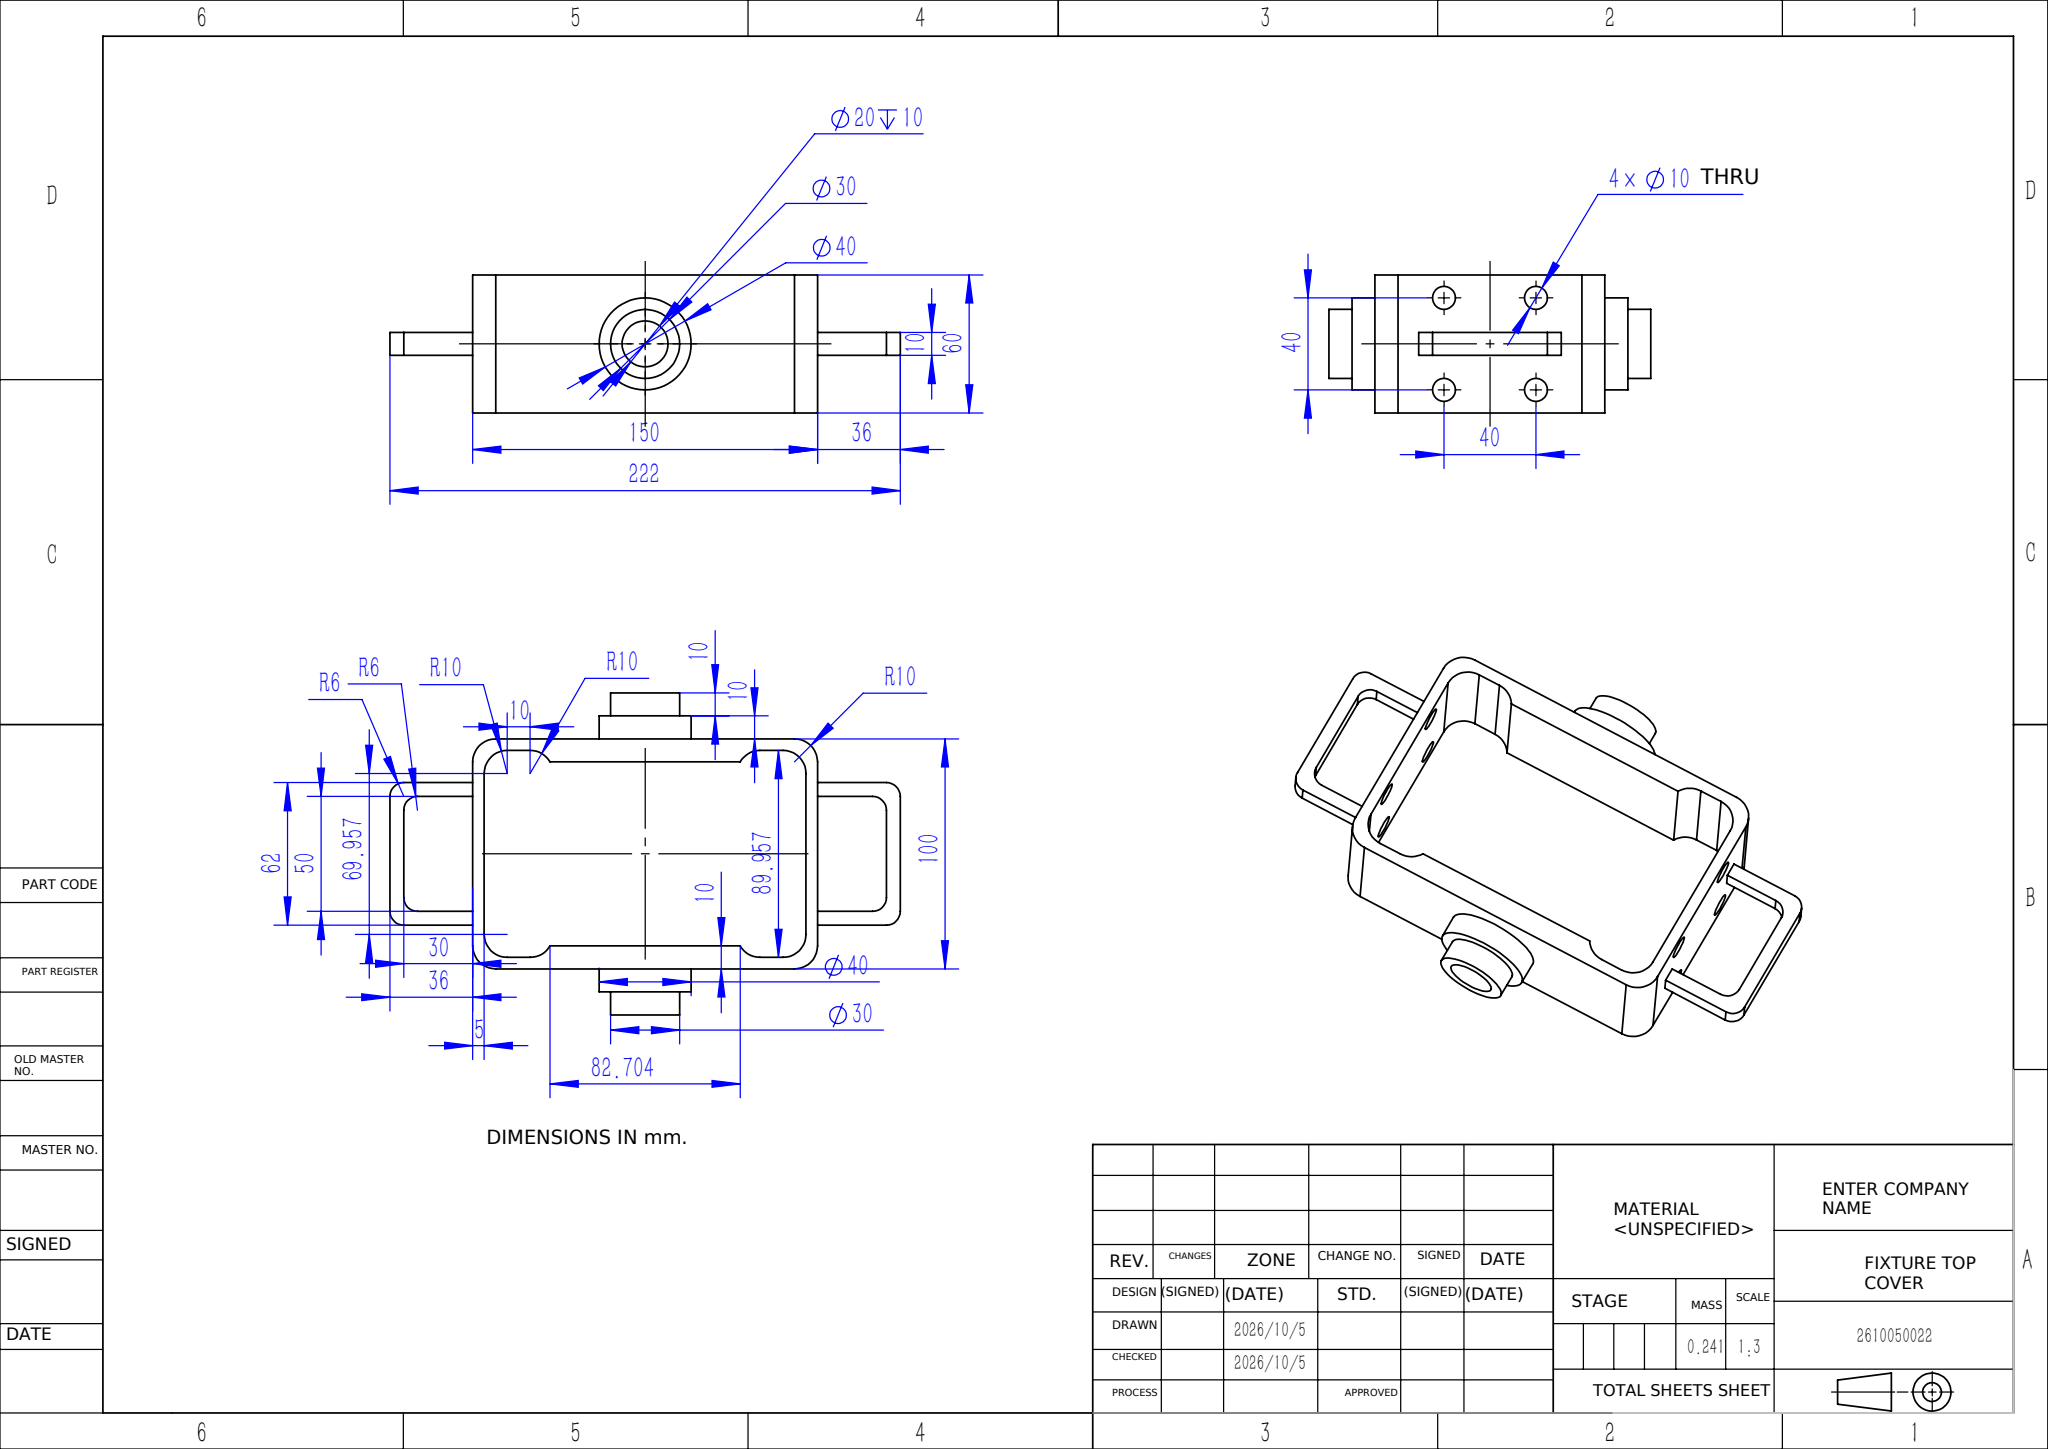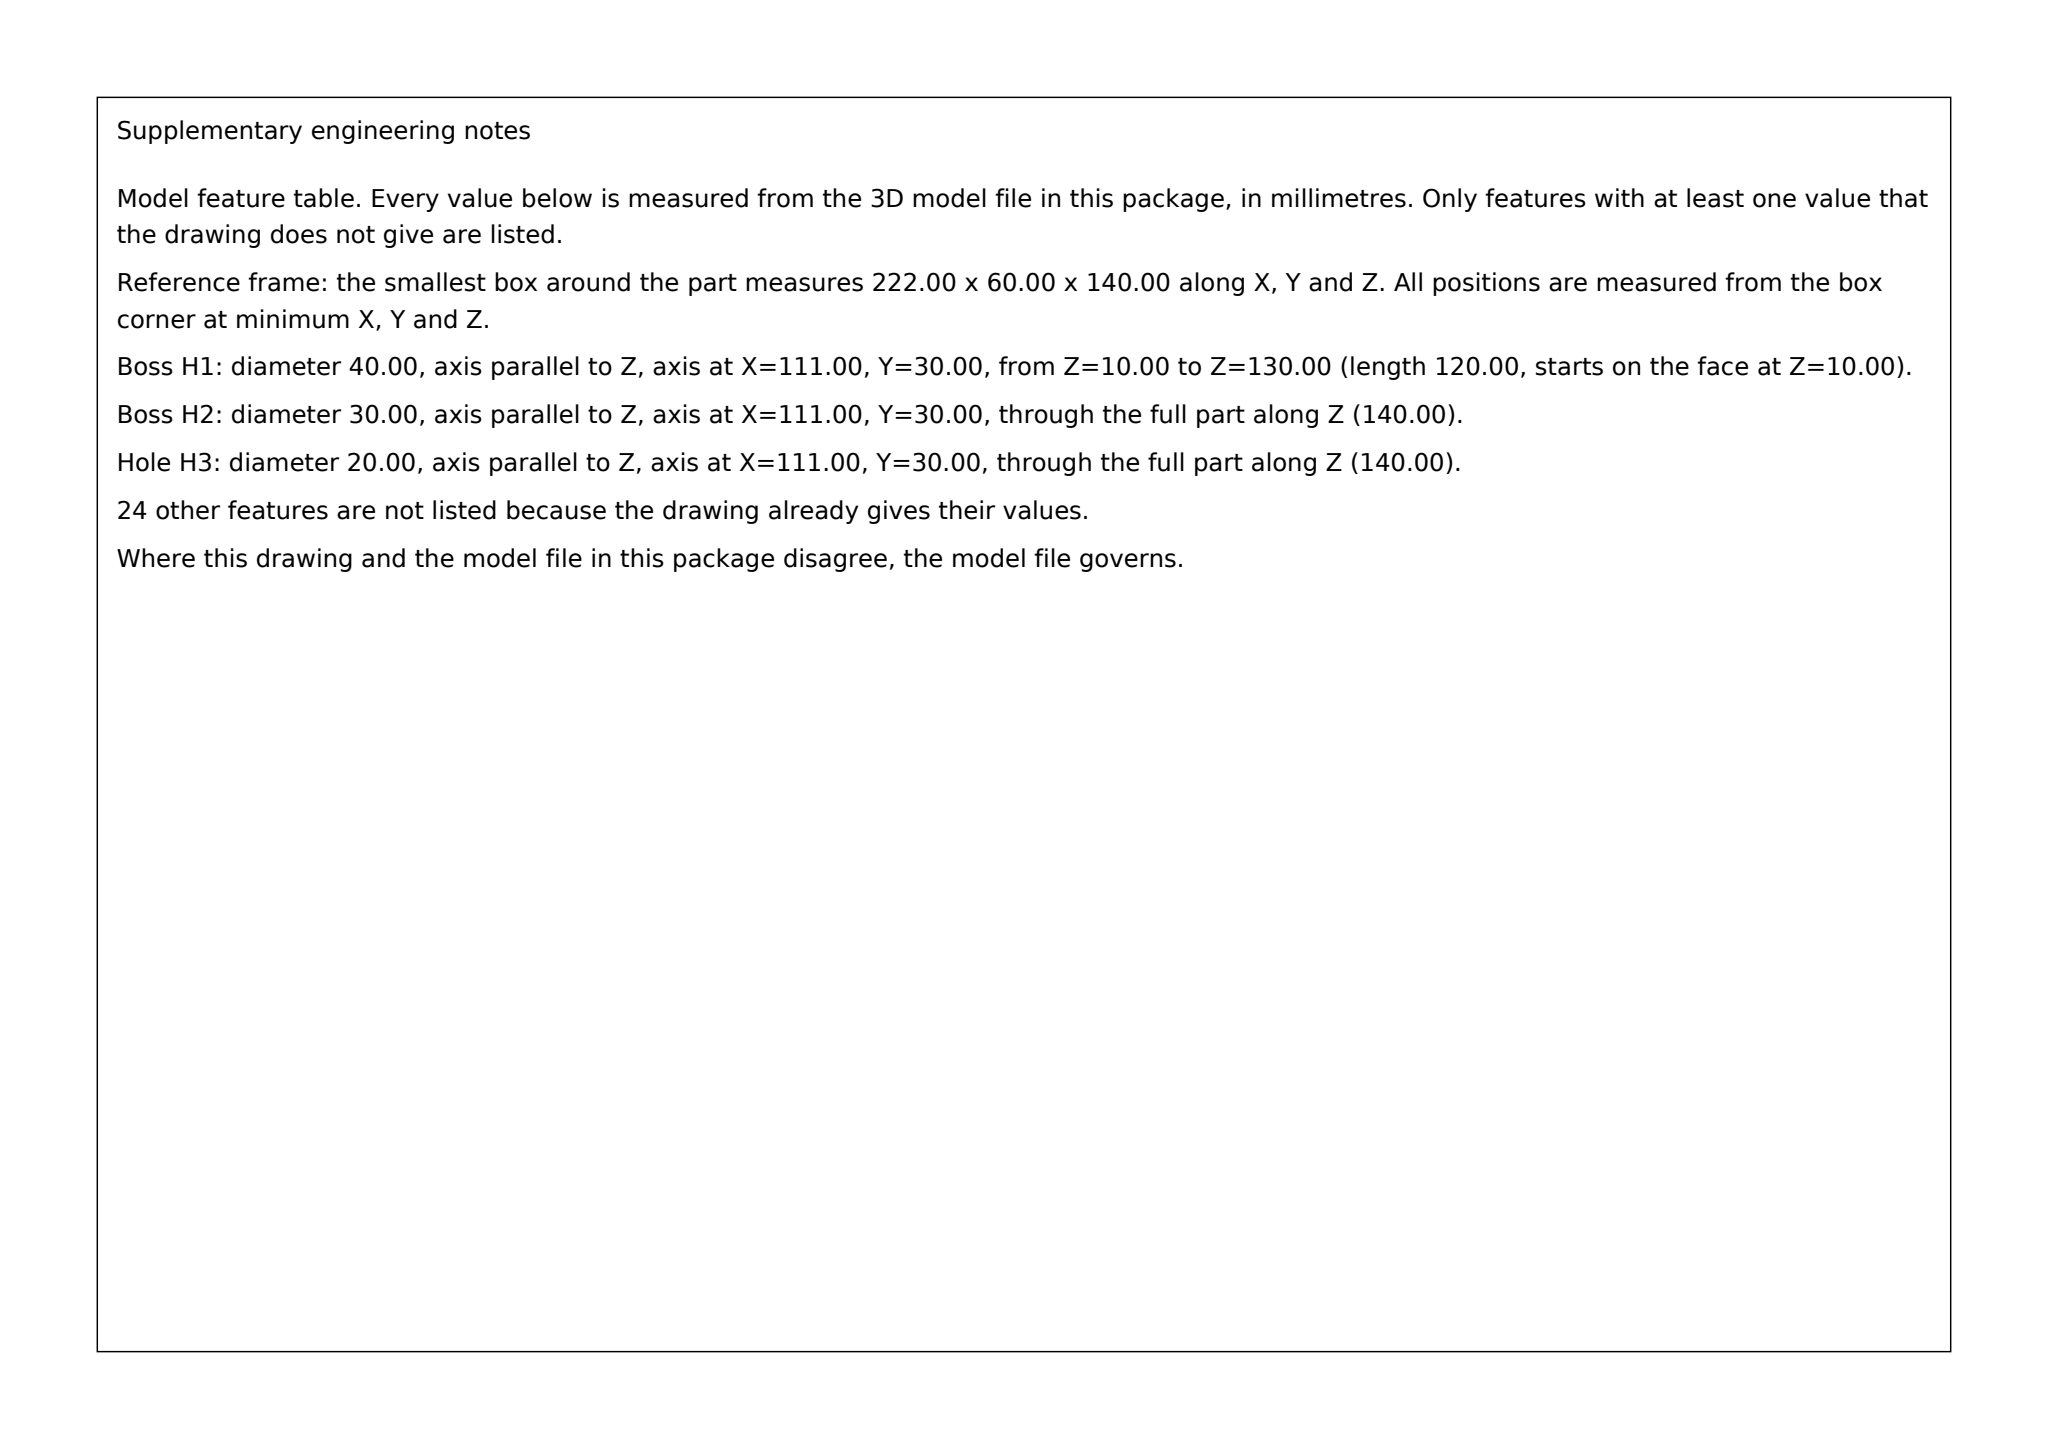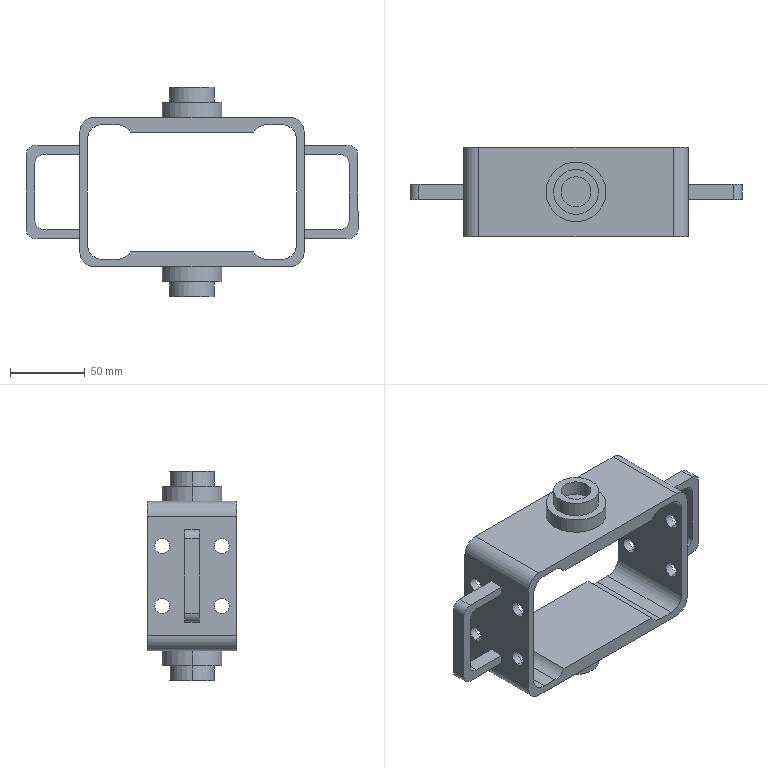Part | SolidWorks | mm | 1 solid | 84 faces | box 222 x 60 x 140 mm | volume 241262 mm3 | cylinder 48 | plane 36 | commonest cylinder face diameters 10 x16 20 x16 12 x8 30 x4 40 x4